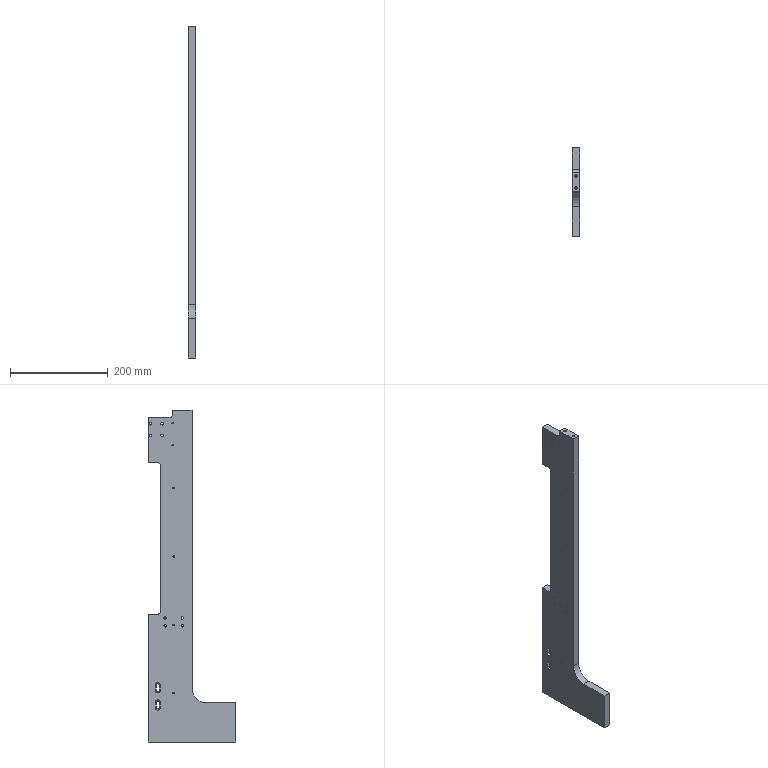Component | SolidWorks | 30-27A-1 | 1 solid | 110 faces | box 15 x 180 x 680 mm | volume 886285 mm3 | cylinder 66 | plane 32 | cone 12 | commonest cylinder face diameters 5 x18 5.5 x8 9.5 x8 3.3 x8 11 x6 6.6 x6 3 x4 10 x3
build123d program:
from build123d import *

# Parameters (mm, degrees)
EXTRUDE1_DEPTH                                    = 15
M4_TAPPED_HOLE3_D                                 = 3.3
LINEAR_PATTERN1_COUNT                             = 5
LINEAR_PATTERN1_PITCH                             = 140
M8_TAPPED_HOLE1_D                                 = 8.1
M8_TAPPED_HOLE1_DEPTH                             = 36.25
M8_TAPPED_HOLE1_TIP                               = 2.433
M6_TAPPED_HOLE3_D                                 = 5
M6_TAPPED_HOLE3_DEPTH                             = 17
M6_TAPPED_HOLE3_TIP                               = 1.502
M6_TAPPED_HOLE1_D                                 = 5
M6_TAPPED_HOLE1_DEPTH                             = 17
M6_TAPPED_HOLE1_TIP                               = 1.502
SKETCH46_W                                        = 310
SKETCH46_H                                        = 25
CUT_EXTRUDE1_DEPTH                                = 704.58
FILLET1_R                                         = 5
M5_SOCKET_HEAD_CAP_SCREW_COUNTERBORE2_D           = 5.5
M5_SOCKET_HEAD_CAP_SCREW_COUNTERBORE2_CBORE_D     = 9.5
M5_SOCKET_HEAD_CAP_SCREW_COUNTERBORE2_CBORE_DEPTH = 5.5
M6_TAPPED_HOLE2_D                                 = 5
CUT_EXTRUDE4_DEPTH                                = 704.58
CUT_EXTRUDE8_DEPTH                                = 6
SKETCH54_R                                        = 1.5
CUT_EXTRUDE5_DEPTH                                = 704.58
CUT_EXTRUDE7_DEPTH                                = 2
CUT_EXTRUDE9_DEPTH                                = 704.58


with BuildPart() as part:
    # Sketch1 → Extrude1 (new body)
    with BuildSketch(Plane.XY):
        with BuildLine():
            Line((0, 0), (0, 180))
            Line((0, 180), (680, 180))
            Line((680, 180), (680, 90))
            Line((680, 90), (110, 90))
            ThreePointArc((110, 90), (88.787, 81.213), (80, 60))
            Line((80, 60), (80, 0))
            Line((80, 0), (0, 0))
        make_face()
    extrude(amount=EXTRUDE1_DEPTH)

    # M4 Tapped Hole3 (through all)
    with Locations(Plane.XY.offset(15)):
        with Locations((100, 127.5)):
            m4_tapped_hole3 = Hole(M4_TAPPED_HOLE3_D / 2)

    # Linear Pattern1: M4 Tapped Hole3 ×5, 1 skipped
    with Locations(*[(i * LINEAR_PATTERN1_PITCH, 0, 0) for i in range(1, LINEAR_PATTERN1_COUNT) if i not in (4,)]):
        add(m4_tapped_hole3, mode=Mode.SUBTRACT)

    # M8 Tapped Hole1
    with Locations(Plane(origin=(0, 180, 0), x_dir=(-1, 0, 0), z_dir=(0, 1, 0))):
        with Locations((-50, 7.5)):
            Hole(M8_TAPPED_HOLE1_D / 2, depth=M8_TAPPED_HOLE1_DEPTH)
            with Locations((0, 0, -(M8_TAPPED_HOLE1_DEPTH + M8_TAPPED_HOLE1_TIP / 2))):  # 118° drill point
                Cone(0, M8_TAPPED_HOLE1_D / 2, M8_TAPPED_HOLE1_TIP, mode=Mode.SUBTRACT)

    # M6 Tapped Hole3
    with Locations(Plane(origin=(680, 0, 0), x_dir=(0, 0, -1), z_dir=(1, 0, 0))):
        with Locations((-7.5, 122), (-7.5, 98)):
            Hole(M6_TAPPED_HOLE3_D / 2, depth=M6_TAPPED_HOLE3_DEPTH)
            with Locations((0, 0, -(M6_TAPPED_HOLE3_DEPTH + M6_TAPPED_HOLE3_TIP / 2))):  # 118° drill point
                Cone(0, M6_TAPPED_HOLE3_D / 2, M6_TAPPED_HOLE3_TIP, mode=Mode.SUBTRACT)

    # M6 Tapped Hole1
    with Locations(Plane.ZY):
        with Locations((7.5, 90), (7.5, 15), (7.5, 165)):
            Hole(M6_TAPPED_HOLE1_D / 2, depth=M6_TAPPED_HOLE1_DEPTH)
            with Locations((0, 0, -(M6_TAPPED_HOLE1_DEPTH + M6_TAPPED_HOLE1_TIP / 2))):  # 118° drill point
                Cone(0, M6_TAPPED_HOLE1_D / 2, M6_TAPPED_HOLE1_TIP, mode=Mode.SUBTRACT)

    # Sketch46 → Cut-Extrude1 (cut, through all)
    with BuildSketch(Plane.XY.offset(15)):
        with Locations((417, 167.5)):
            Rectangle(SKETCH46_W, SKETCH46_H)
    extrude(amount=-CUT_EXTRUDE1_DEPTH, mode=Mode.SUBTRACT)

    # Fillet1
    fillet1_edges = [part.edges().sort_by_distance(p)[0] for p in [
        (572, 155, 7.5),
        (262, 155, 7.5),
    ]]
    fillet(fillet1_edges, radius=FILLET1_R)

    # M5 Socket Head Cap Screw Counterbore2 (through all)
    with Locations(Plane(origin=(17.587, 3.323, 0), x_dir=(1, 0, 0), z_dir=(0, 0, -1))):
        with Locations((634.413, -171.677), (610.413, -171.677), (634.413, -147.677), (610.413, -147.677)):
            CounterBoreHole(M5_SOCKET_HEAD_CAP_SCREW_COUNTERBORE2_D / 2, M5_SOCKET_HEAD_CAP_SCREW_COUNTERBORE2_CBORE_D / 2, M5_SOCKET_HEAD_CAP_SCREW_COUNTERBORE2_CBORE_DEPTH)

    # M6 Tapped Hole2 (through all)
    with Locations(Plane.XY.offset(15)):
        with Locations((238, 145), (254, 145), (238, 110), (254, 110)):
            Hole(M6_TAPPED_HOLE2_D / 2)

    # Sketch60 → Cut-Extrude4 (cut, through all)
    with BuildSketch(Plane.XY.offset(15)):
        with BuildLine():
            Line((71, 163.3), (81, 163.3))
            ThreePointArc((81, 163.3), (84.3, 160), (81, 156.7))
            Line((81, 156.7), (71, 156.7))
            ThreePointArc((71, 156.7), (67.7, 160), (71, 163.3))
        make_face()
        with BuildLine():
            Line((116, 156.7), (106, 156.7))
            ThreePointArc((106, 156.7), (102.7, 160), (106, 163.3))
            Line((106, 163.3), (116, 163.3))
            ThreePointArc((116, 163.3), (119.3, 160), (116, 156.7))
        make_face()
    extrude(amount=-CUT_EXTRUDE4_DEPTH, mode=Mode.SUBTRACT)

    # Sketch59 → Cut-Extrude8 (cut)
    # profile 1 of 2: a face of its own
    with BuildSketch(Plane.XY.offset(15)):
        with BuildLine():
            Line((71, 154.5), (81, 154.5))
            ThreePointArc((81, 154.5), (86.5, 160), (81, 165.5))
            Line((81, 165.5), (71, 165.5))
            ThreePointArc((71, 165.5), (65.5, 160), (71, 154.5))
        make_face()
        with BuildLine():
            Line((71, 156.7), (81, 156.7))
            ThreePointArc((81, 156.7), (84.3, 160), (81, 163.3))
            Line((81, 163.3), (71, 163.3))
            ThreePointArc((71, 163.3), (67.7, 160), (71, 156.7))
        make_face(mode=Mode.SUBTRACT)
    # profile 2 of 2: a face of its own
    with BuildSketch(Plane.XY.offset(15)):
        with BuildLine():
            Line((106, 154.5), (116, 154.5))
            ThreePointArc((116, 154.5), (121.5, 160), (116, 165.5))
            Line((116, 165.5), (106, 165.5))
            ThreePointArc((106, 165.5), (100.5, 160), (106, 154.5))
        make_face()
        with BuildLine():
            Line((106, 156.7), (116, 156.7))
            ThreePointArc((116, 156.7), (119.3, 160), (116, 163.3))
            Line((116, 163.3), (106, 163.3))
            ThreePointArc((106, 163.3), (102.7, 160), (106, 156.7))
        make_face(mode=Mode.SUBTRACT)
    extrude(amount=-CUT_EXTRUDE8_DEPTH, mode=Mode.SUBTRACT)

    # Sketch54 → Cut-Extrude5 (cut, through all)
    with BuildSketch(Plane.XY.offset(15)):
        with Locations((653, 129.5)):
            Circle(SKETCH54_R)
        with Locations((608, 129.5)):
            Circle(SKETCH54_R)
    extrude(amount=-CUT_EXTRUDE5_DEPTH, mode=Mode.SUBTRACT)

    # Sketch63 → Cut-Extrude7 (cut)
    with BuildSketch(Plane(origin=(0, 0, 0), x_dir=(-1, 0, 0), z_dir=(0, 0, -1))):
        with BuildLine():
            Line((-128.5, 180), (-58.5, 180))
            Line((-58.5, 180), (-58.5, 157))
            ThreePointArc((-58.5, 157), (-59.086, 155.586), (-60.5, 155))
            Line((-60.5, 155), (-126.5, 155))
            ThreePointArc((-126.5, 155), (-127.914, 155.586), (-128.5, 157))
            Line((-128.5, 157), (-128.5, 180))
        make_face()
    extrude(amount=-CUT_EXTRUDE7_DEPTH, mode=Mode.SUBTRACT)

    # Sketch64 → Cut-Extrude9 (cut, through all)
    with BuildSketch(Plane.XY.offset(15)):
        with BuildLine():
            Line((680, 180), (665, 180))
            Line((665, 180), (665, 135))
            ThreePointArc((665, 135), (666.464, 131.464), (670, 130))
            Line((670, 130), (680, 130))
            Line((680, 130), (680, 180))
        make_face()
    extrude(amount=-CUT_EXTRUDE9_DEPTH, mode=Mode.SUBTRACT)


solid = part.part

# Placed as in the assembly
solid = solid.moved(Location((-854.208, -167.092, 39.188), (0, -90, 0)))